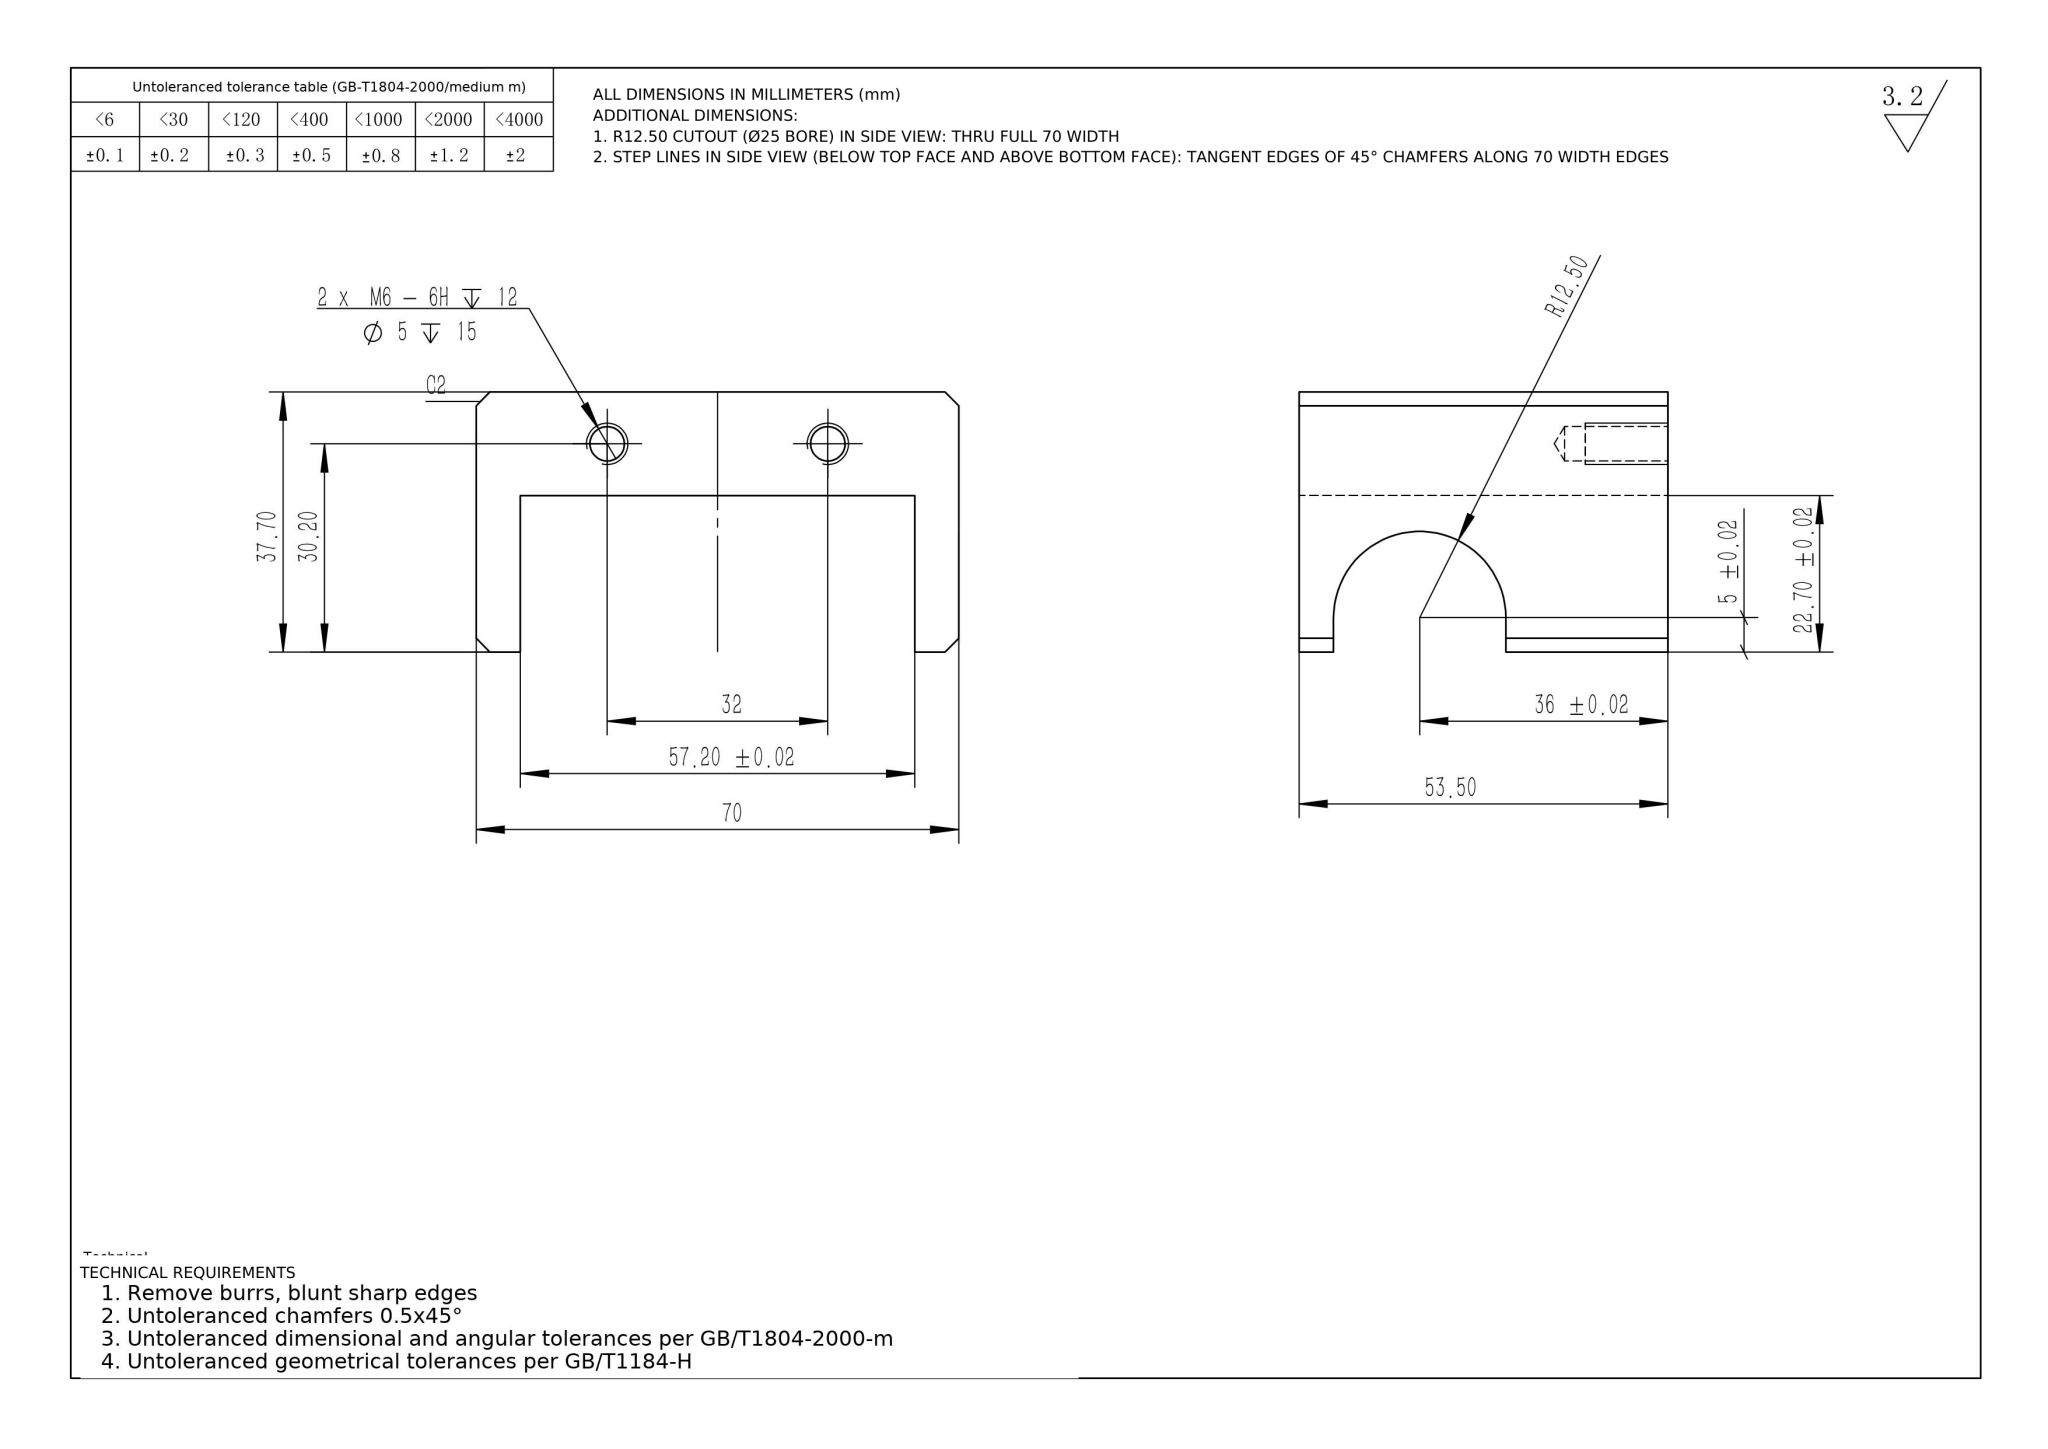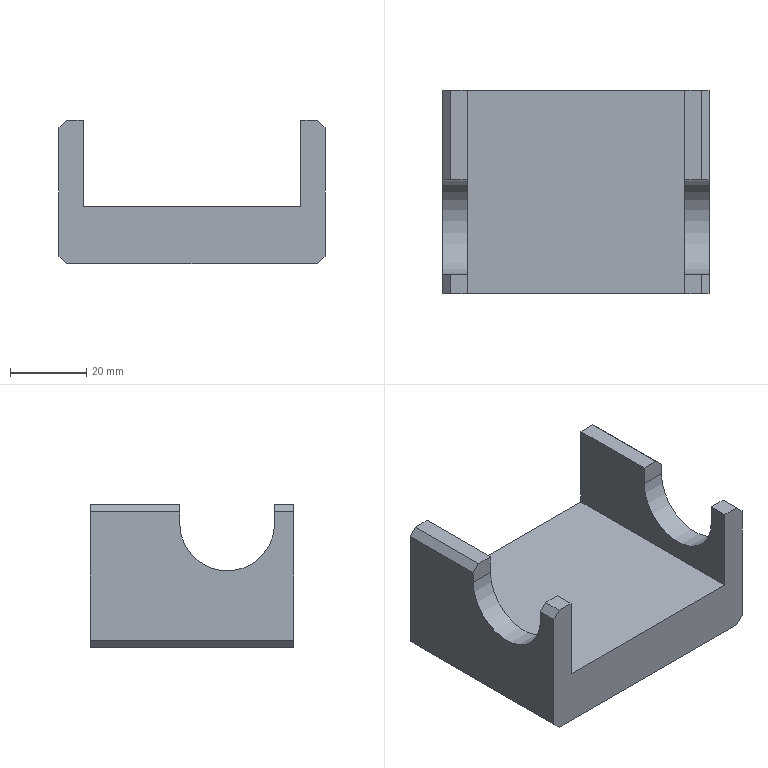Part | NX | mm | 1 solid | 32 faces | box 70 x 53.5 x 37.7 mm | volume 66042 mm3 | plane 22 | cylinder 6 | cone 4 | commonest cylinder face diameters 5 x4 25 x2